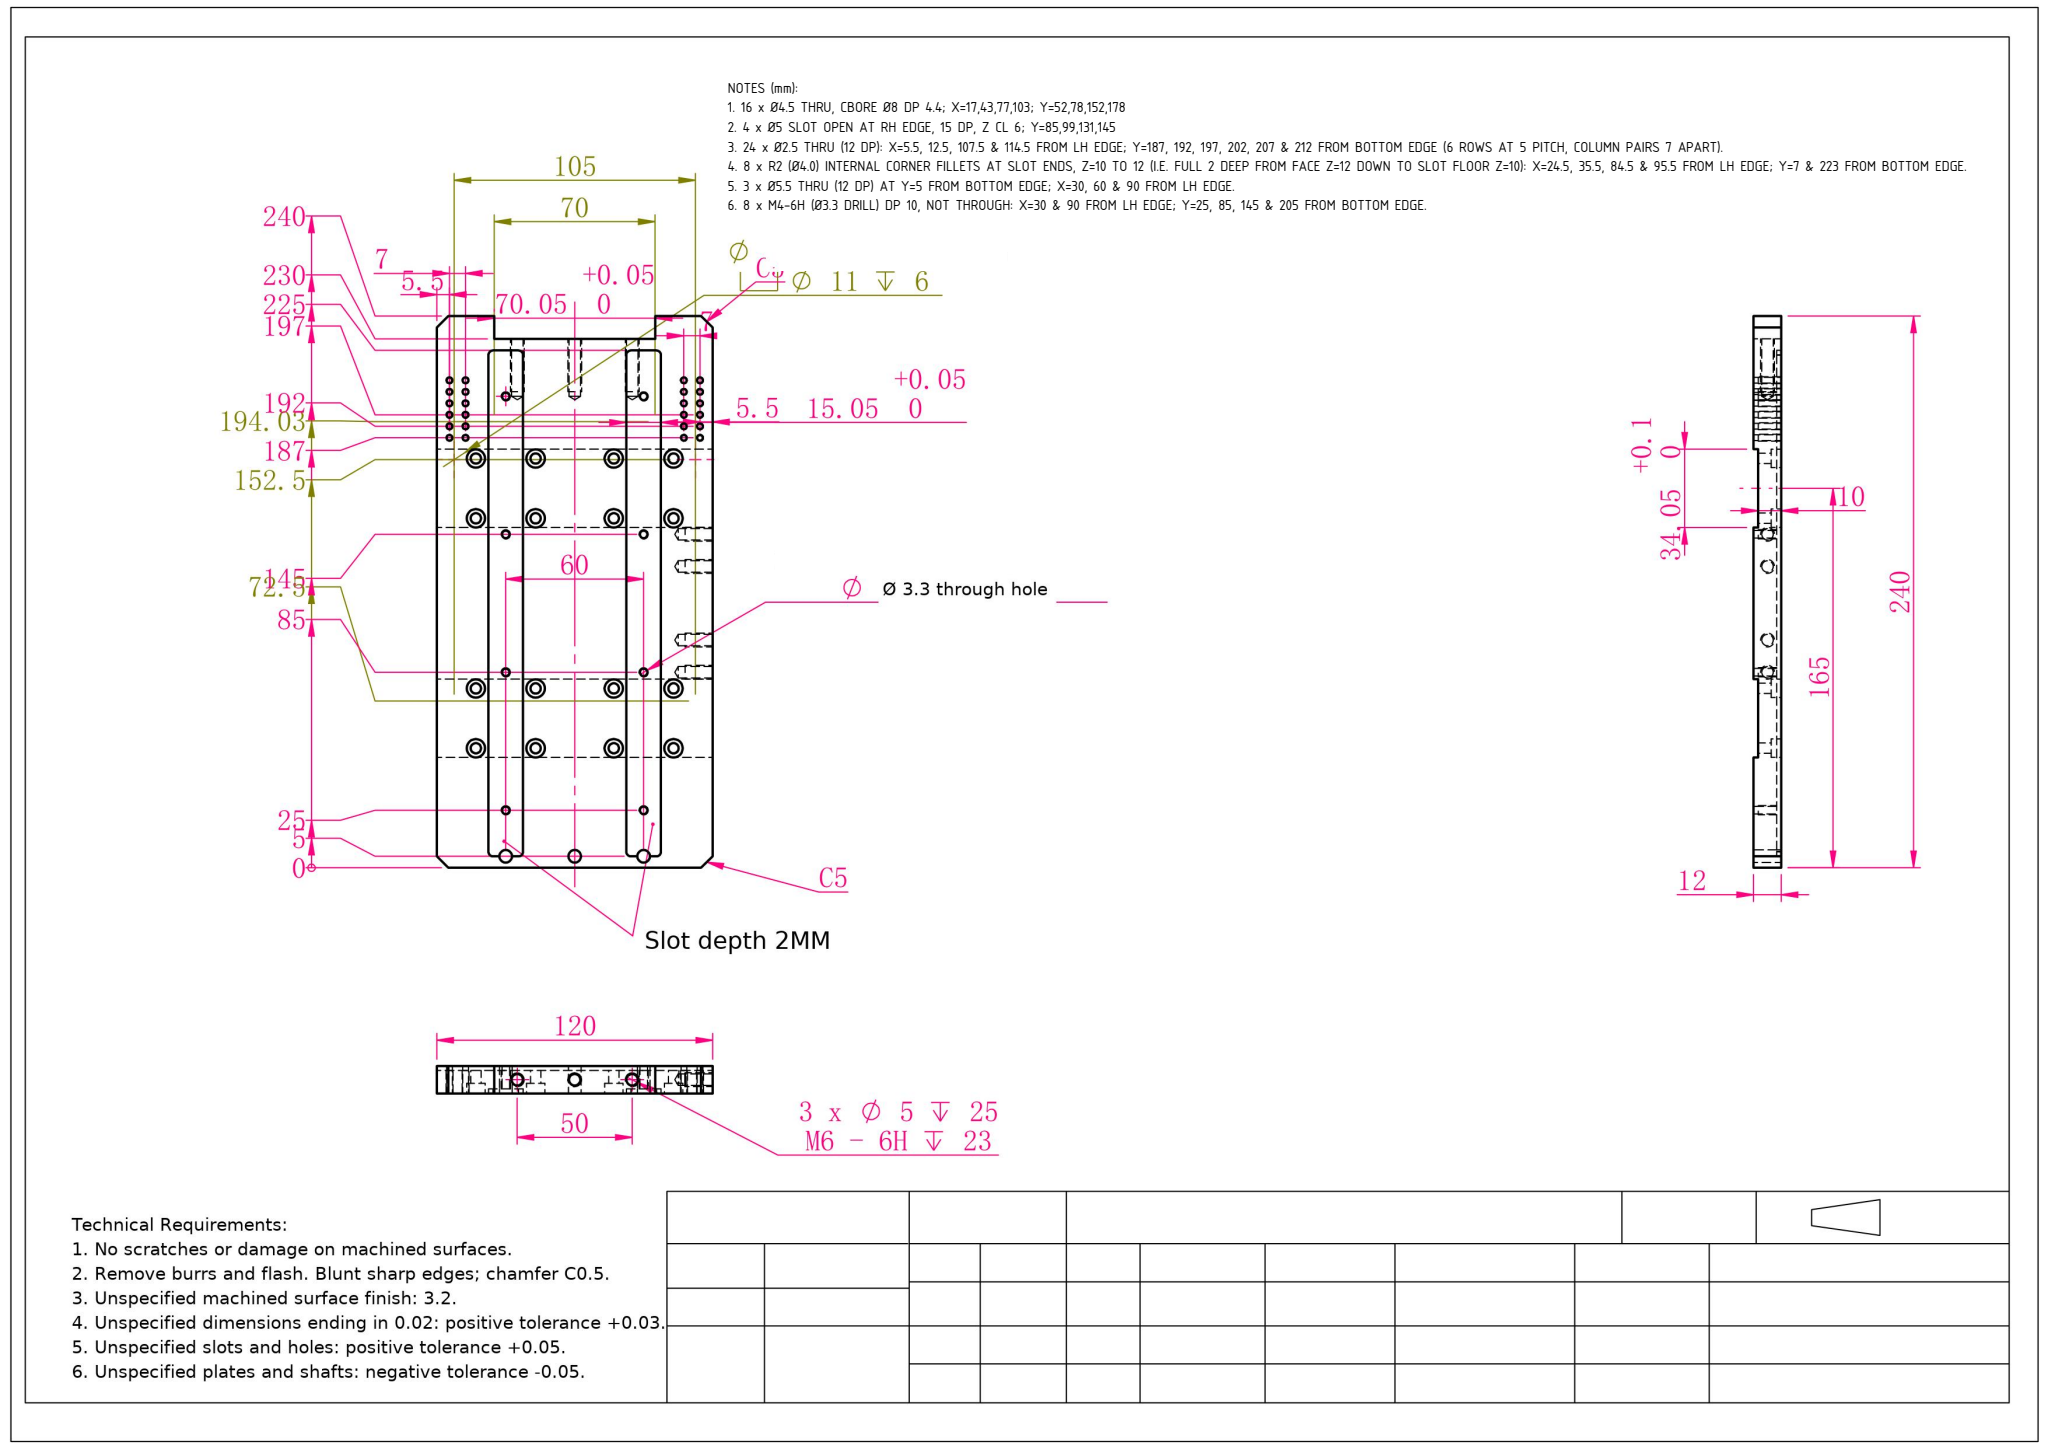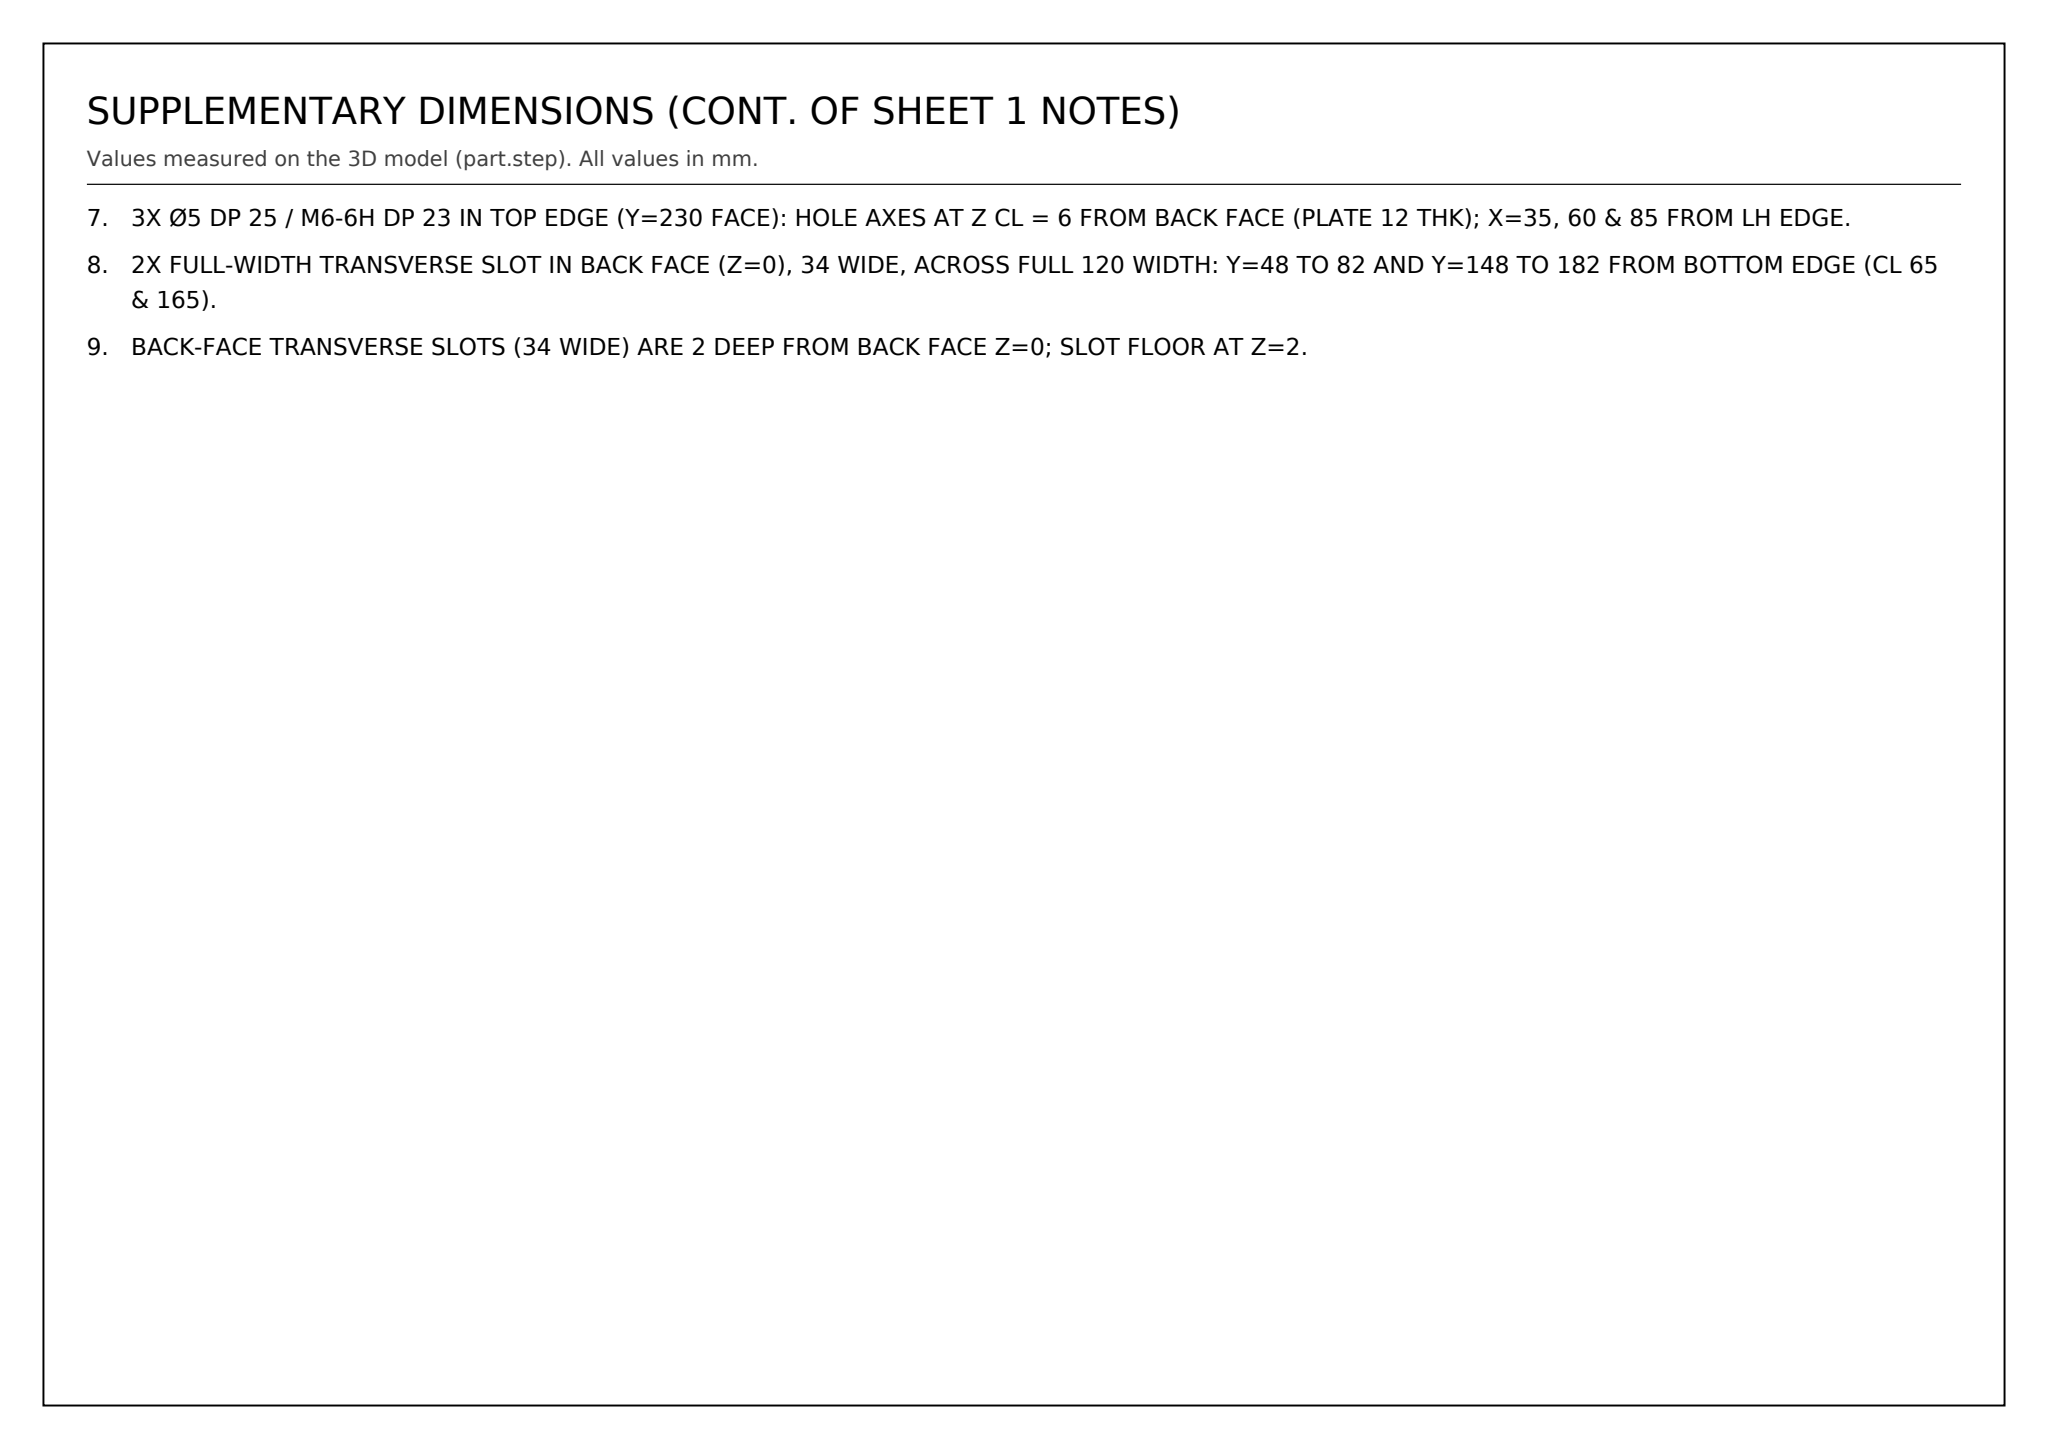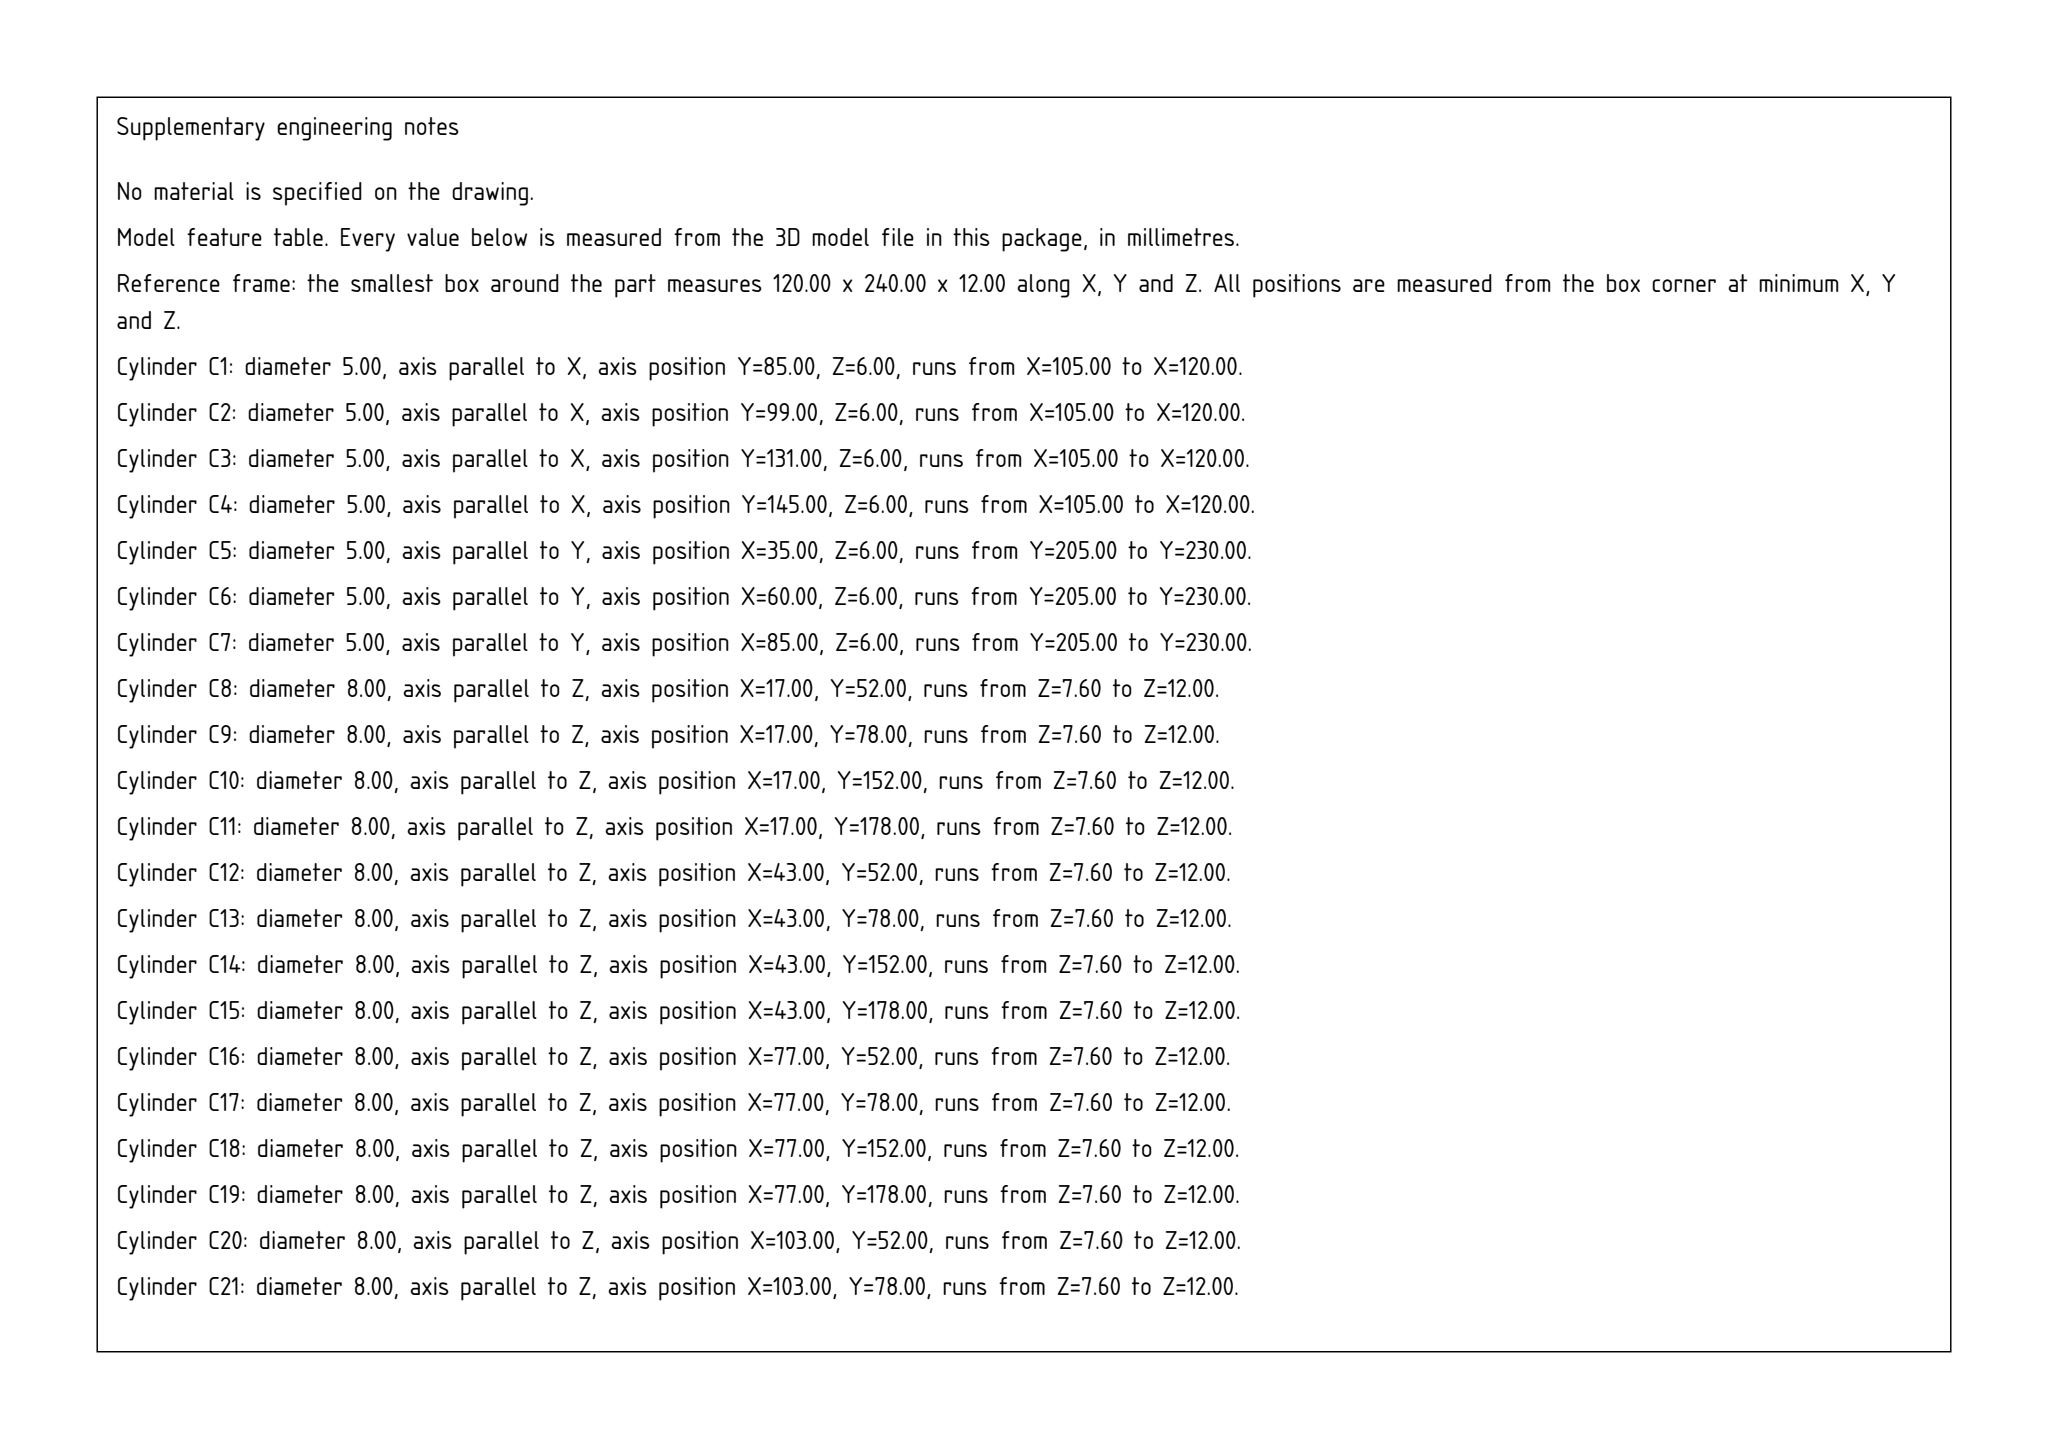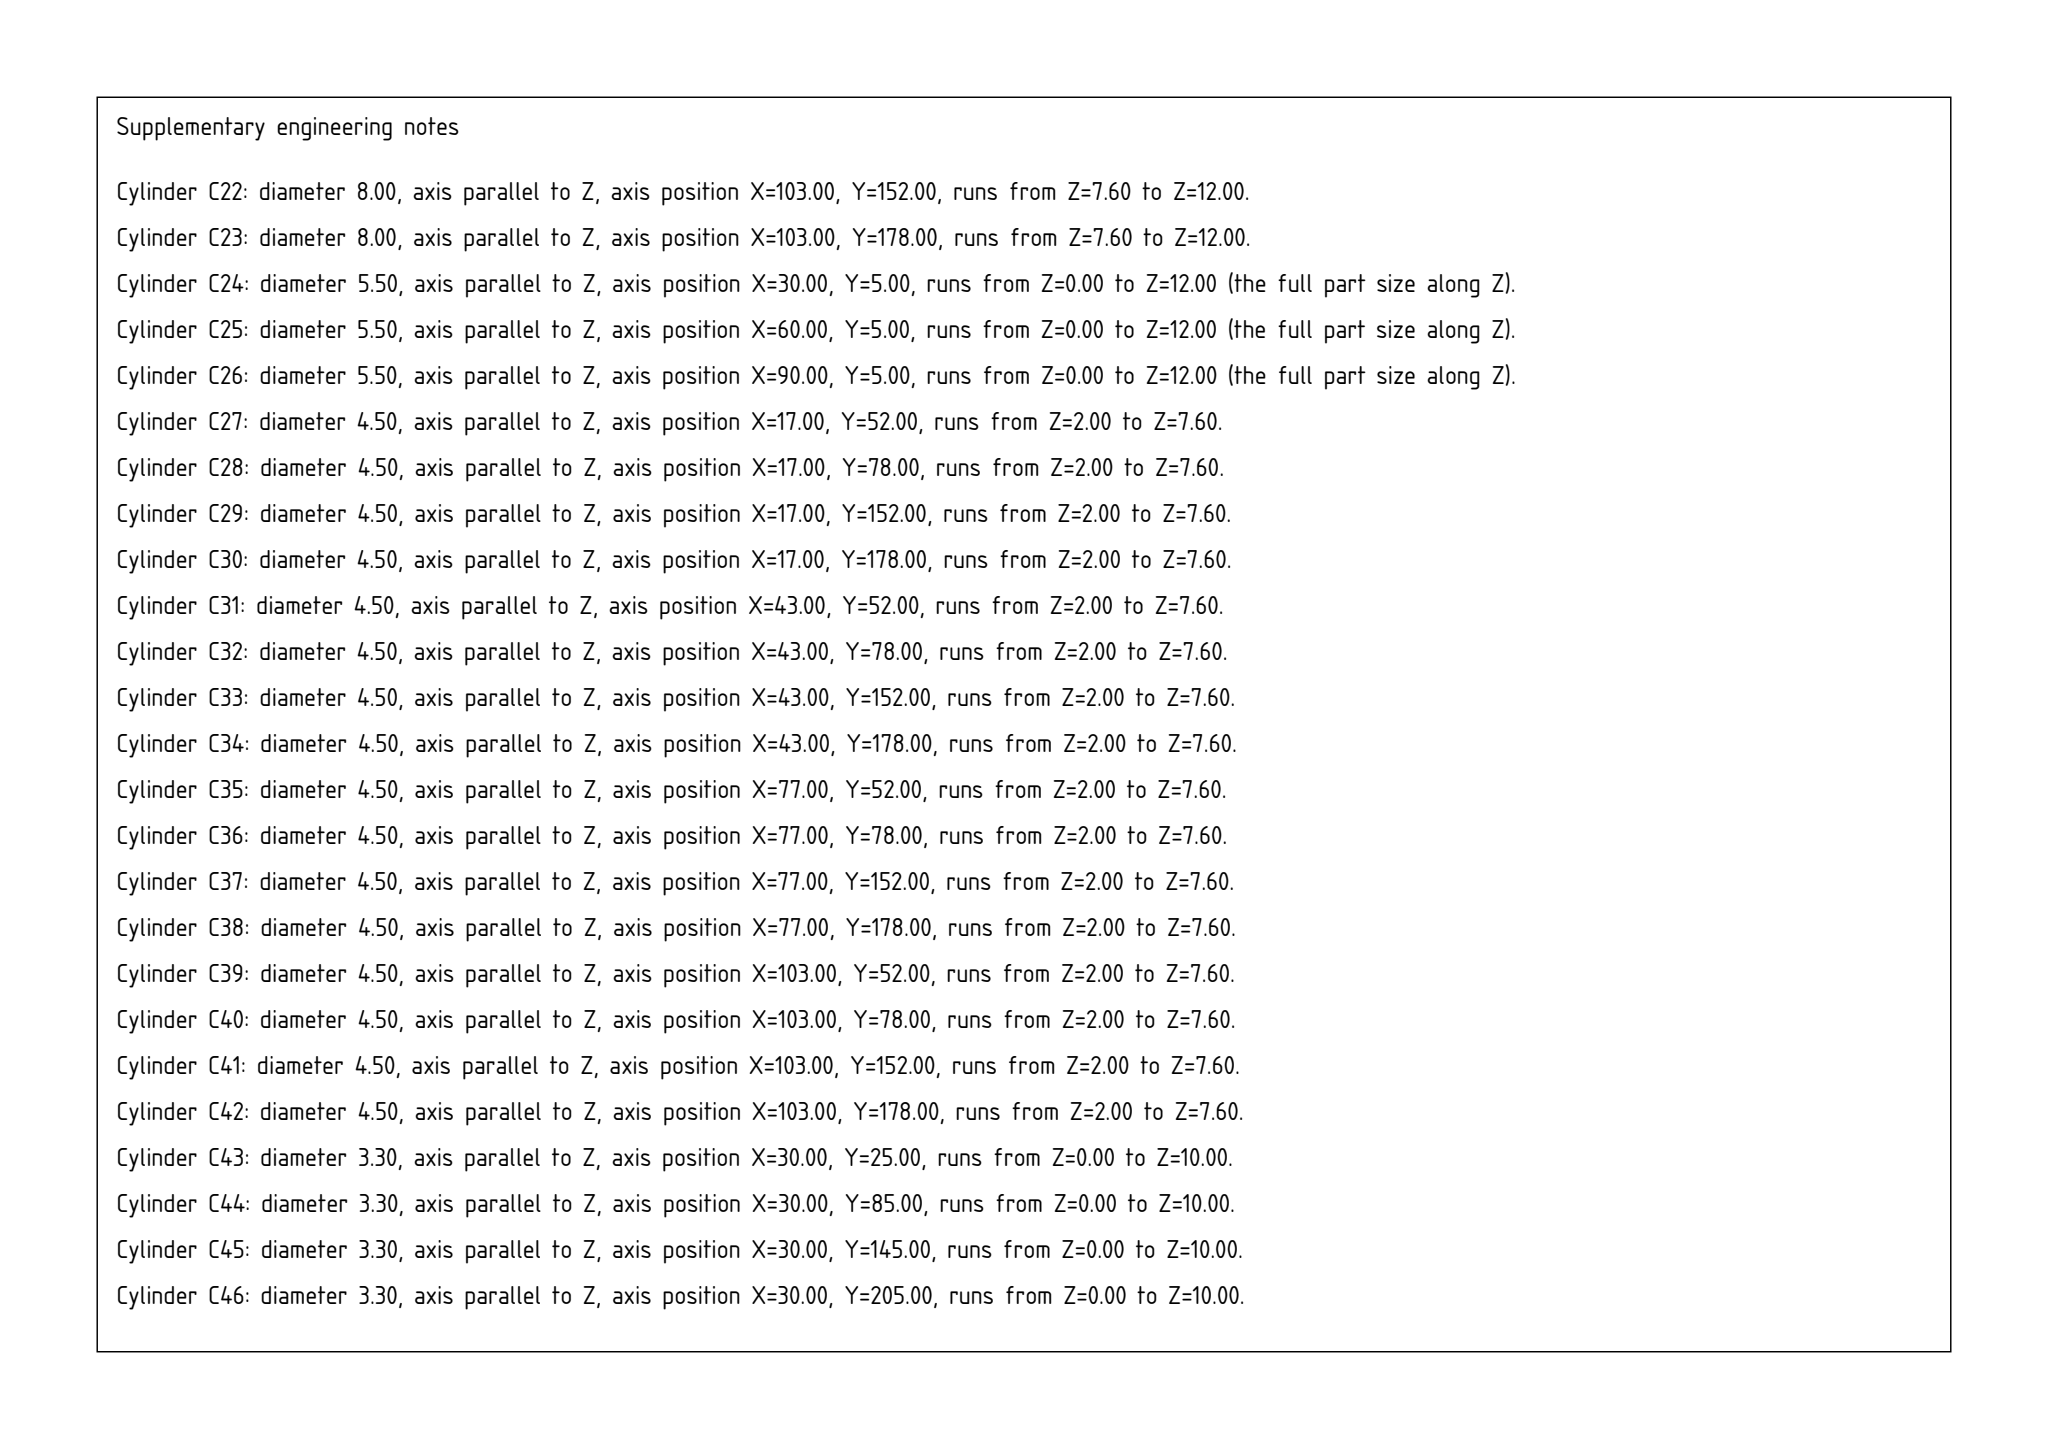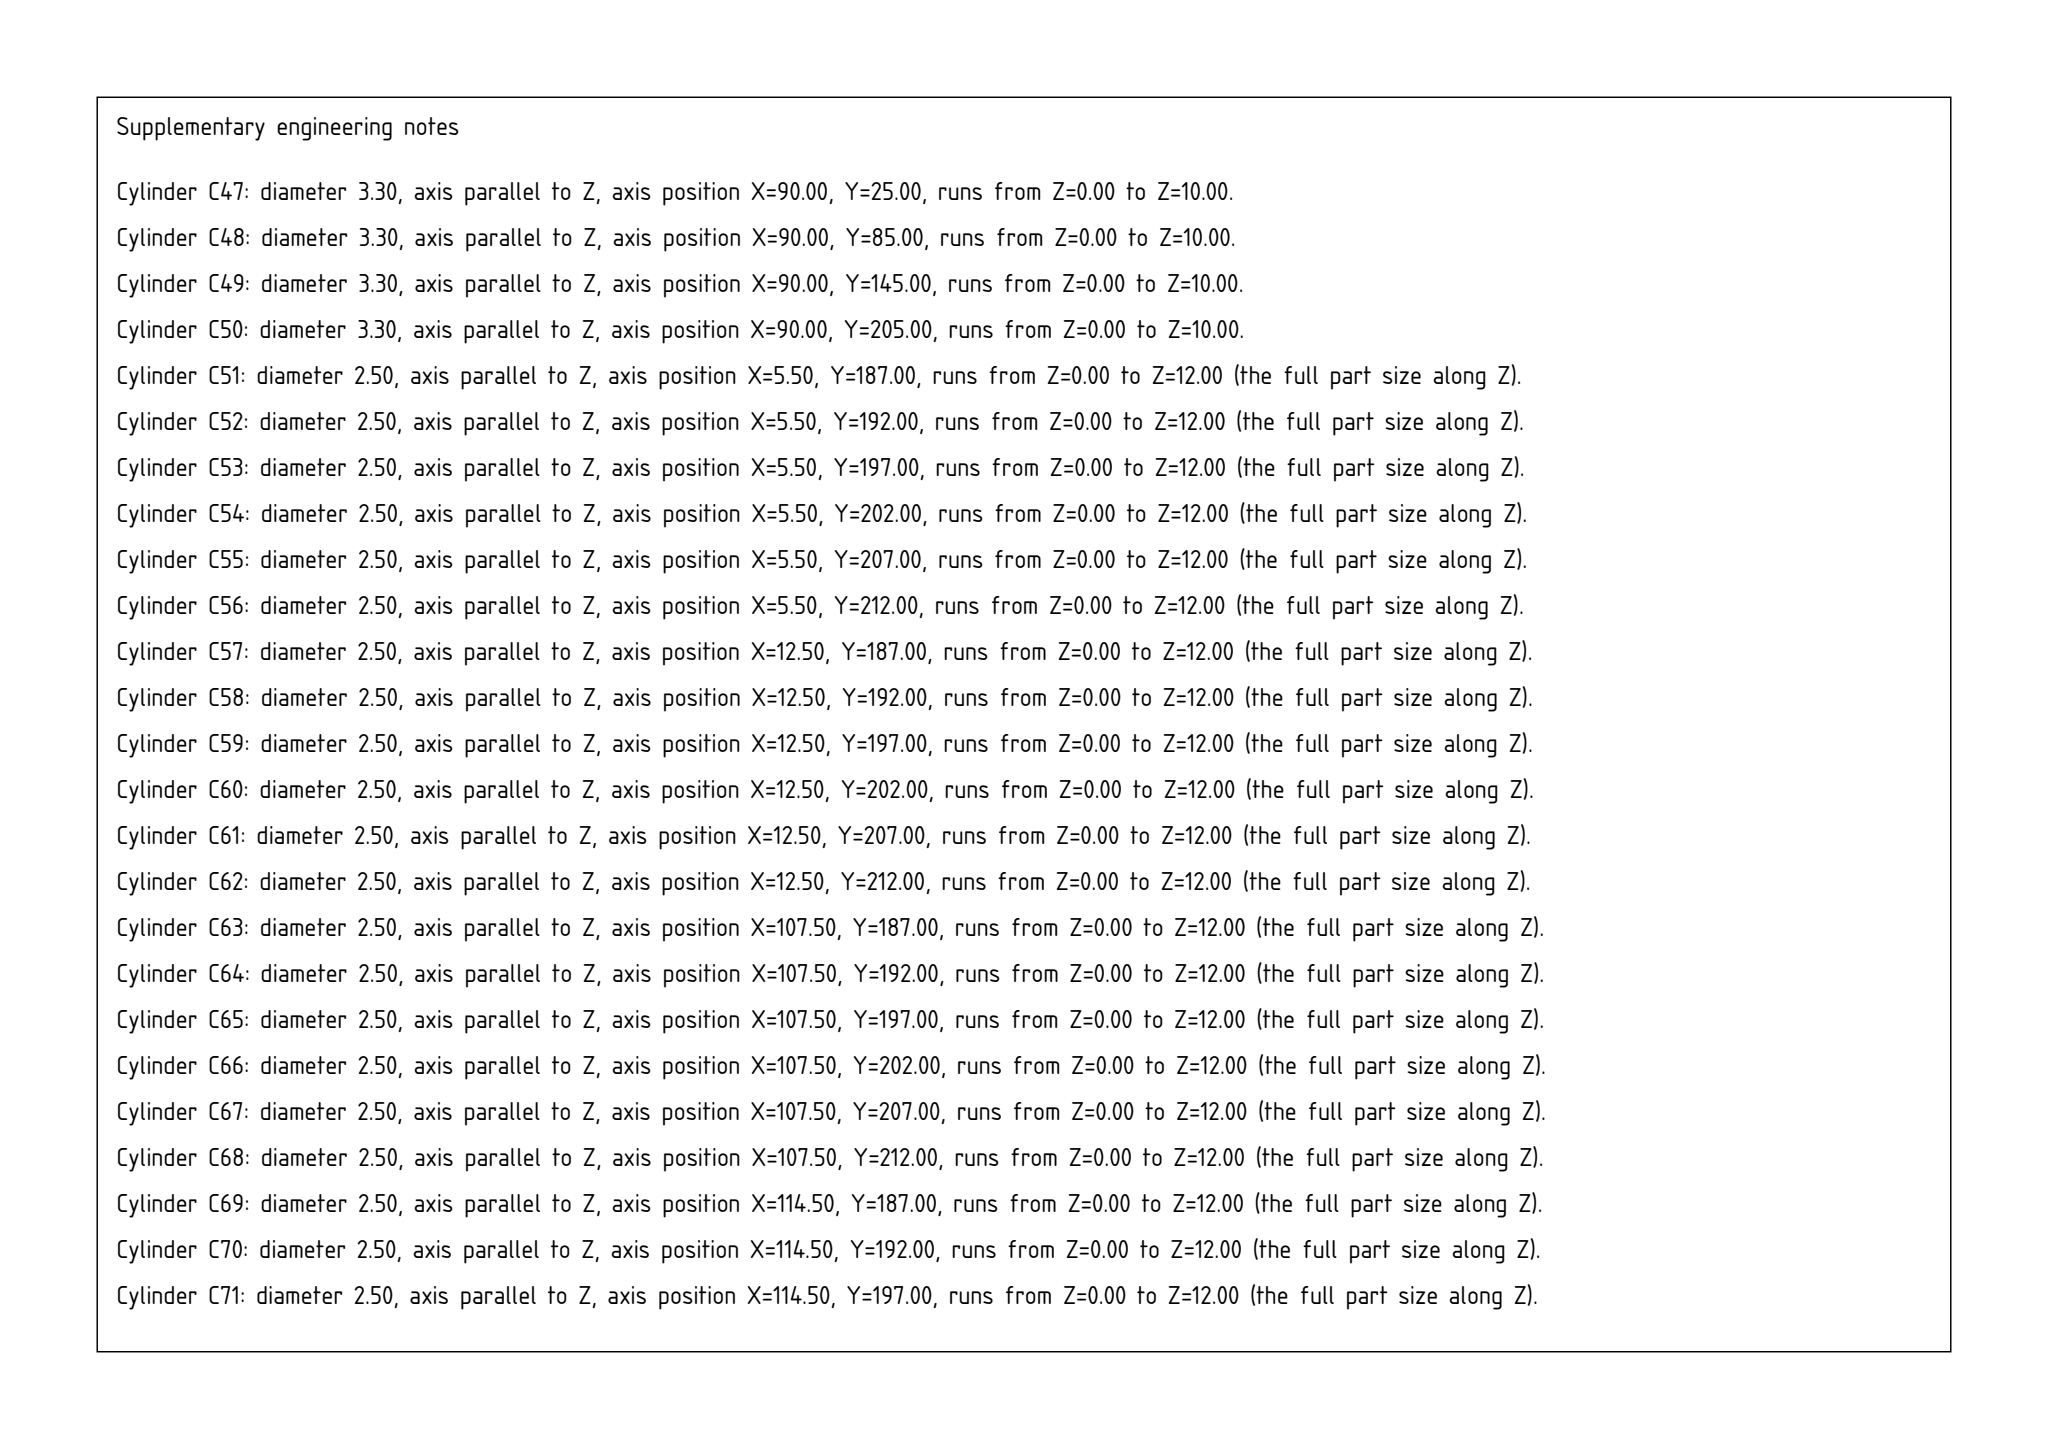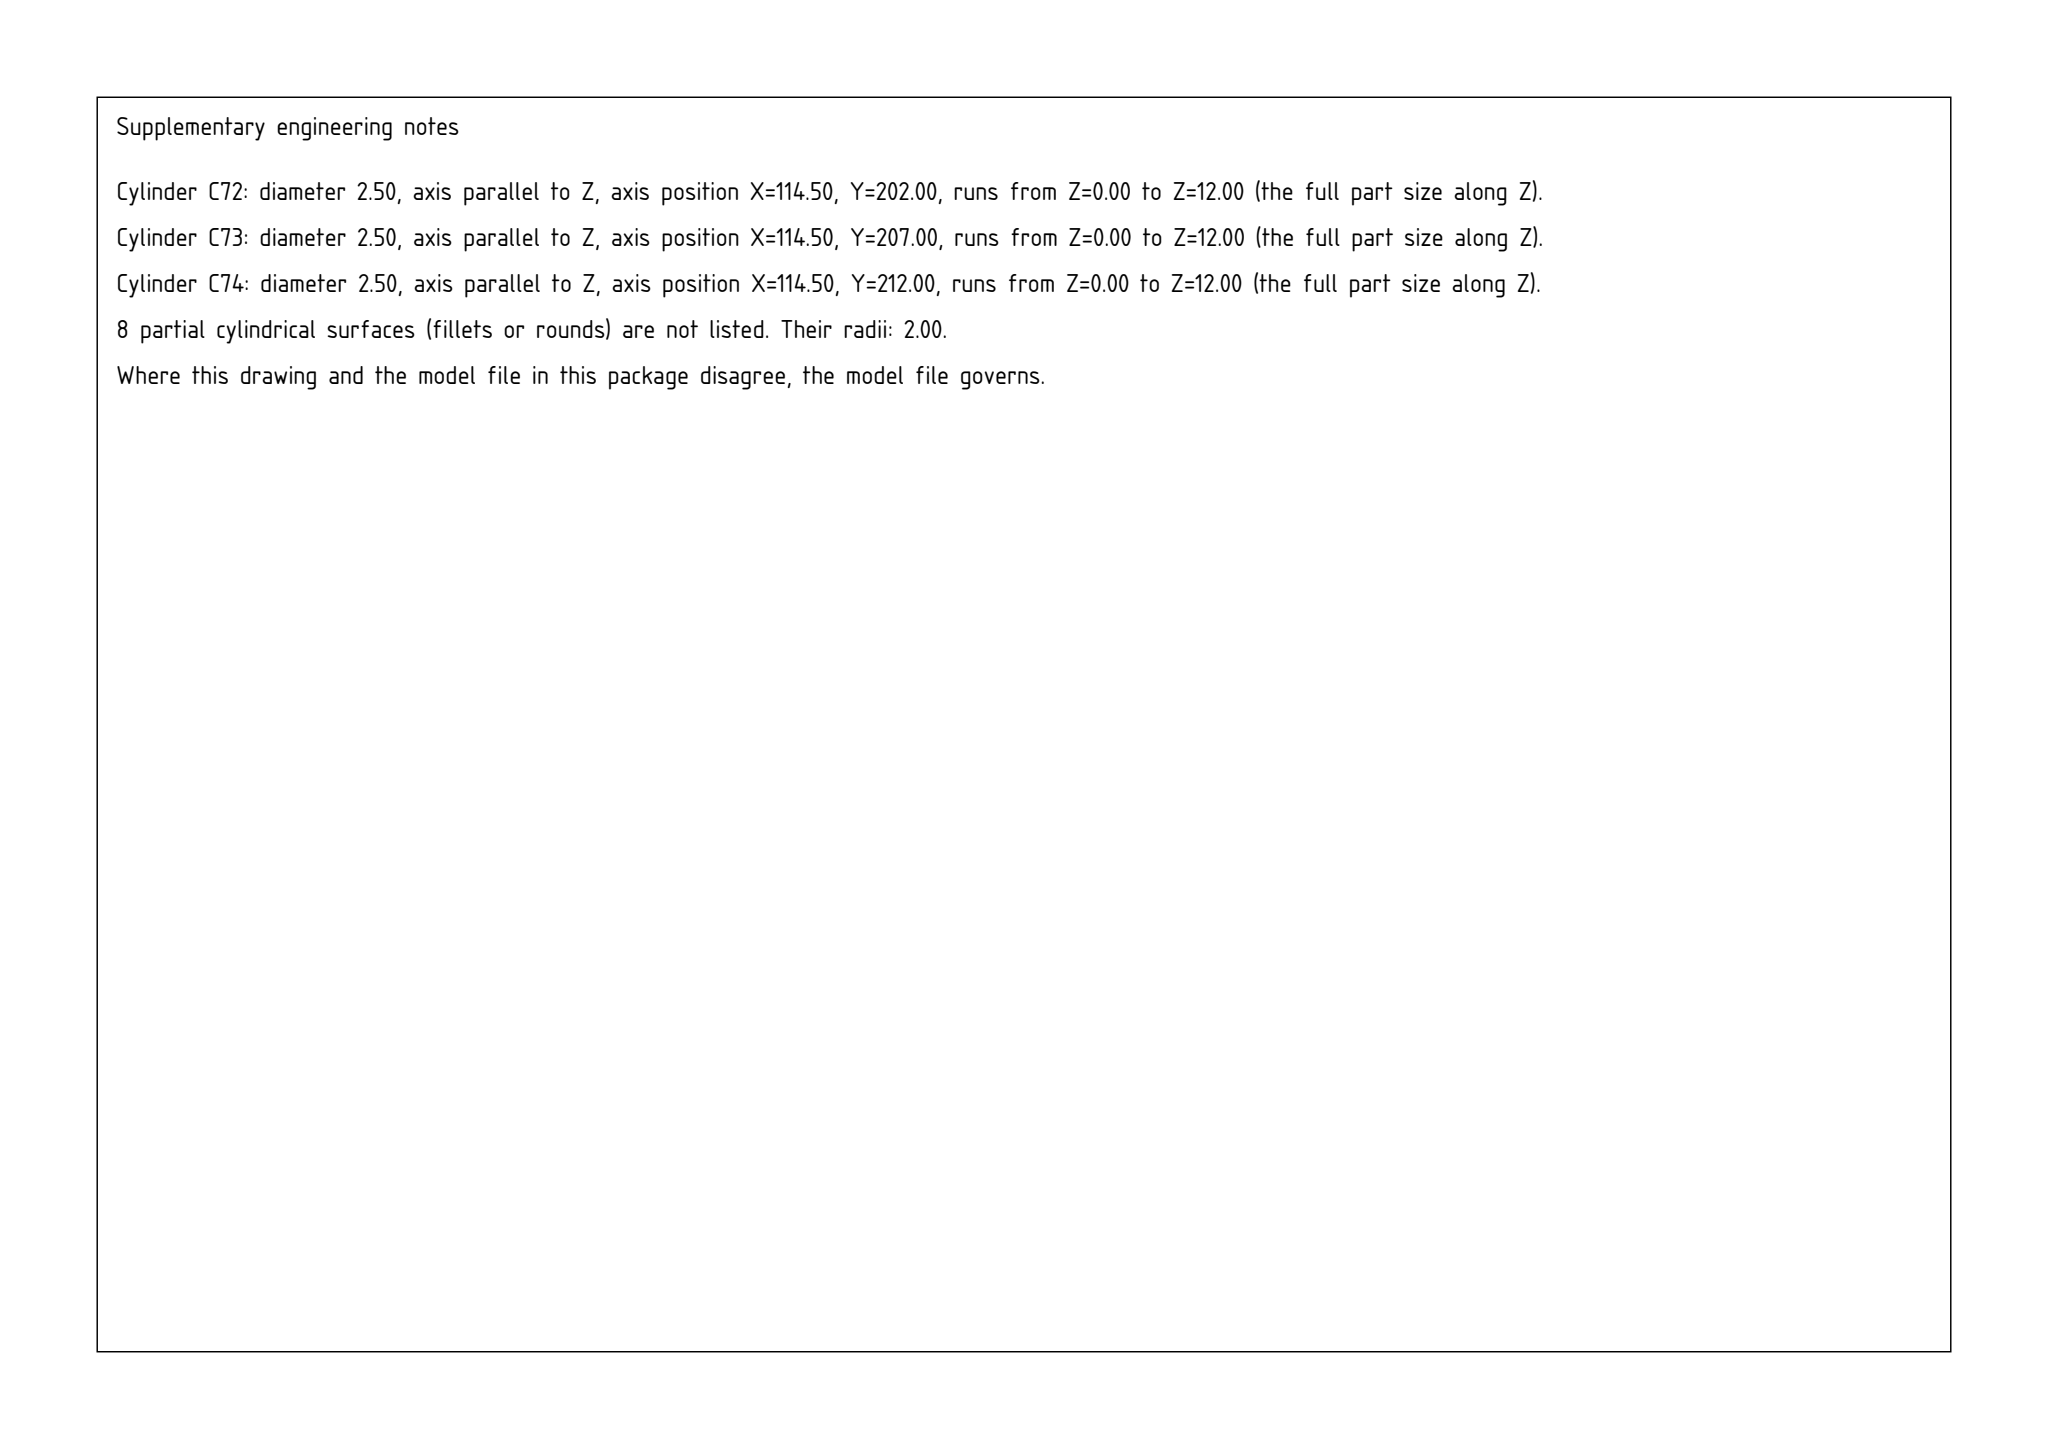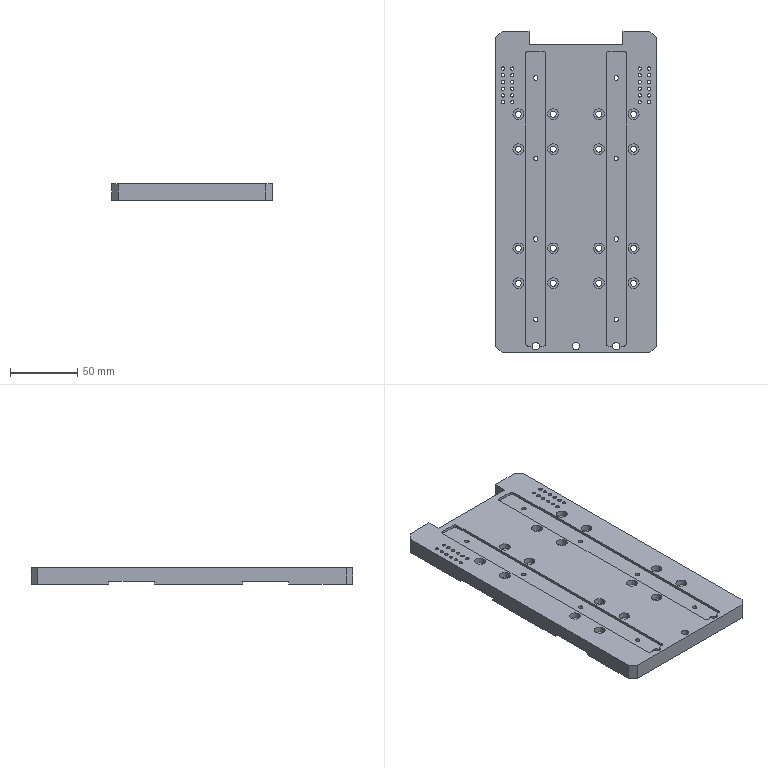Part | SolidWorks | mm | 1 solid | 220 faces | box 120 x 240 x 12 mm | volume 296431 mm3 | cylinder 156 | plane 50 | cone 14 | commonest cylinder face diameters 2.5 x48 8 x32 4.5 x32 3.3 x16 5 x14 4 x8 5.5 x6
Drawing notes:
16 x Ø4.5 THRU, CBORE Ø8 DP 4.4; X=17,43,77,103; Y=52,78,152,178 | from the solid: Cyl Ø4.5 len 5.6 with Ø8 cbore len 4.4 at x=17,43,77,103 and y=52,78,152,178
4 x Ø5 SLOT OPEN AT RH EDGE, 15 DP, Z CL 6; Y=85,99,131,145 | from the solid: Cyl Ø5 axis x len 15 at y=85,99,131,145, z=6; bbox x=120 RH edge
24 x Ø2.5 THRU (12 DP): X=5.5, 12.5, 107.5 & 114.5 FROM LH EDGE; Y=187, 192, 197, 202, 207 & 212 FROM BOTTOM EDGE (6 ROWS AT 5 PITCH, COLUMN PAIRS 7 APART). | from the solid: cylinders dia 2.5, axis z, length 12.0, pos (5.5/12.5/107.5/114.5, 187/192/197/202/207/212)
8 x R2 (Ø4.0) INTERNAL CORNER FILLETS AT SLOT ENDS, Z=10 TO 12 (I.E. FULL 2 DEEP FROM FACE Z=12 DOWN TO SLOT FLOOR Z=10): X=24.5, 35.5, 84.5 & 95.5 FROM LH EDGE; Y=7 & 223 FROM BOTTOM EDGE. | from the solid: cylinders dia 4.0, axis z, 90 deg arcs at (24.5,7),(24.5,223),(35.5,7),(35.5,223),(84.5,7),(84.5,223),(95.5,7),(95.5,223), each from z=10 to z=12; slot floor plane z=10, face z=12
3 x Ø5.5 THRU (12 DP) AT Y=5 FROM BOTTOM EDGE; X=30, 60 & 90 FROM LH EDGE. | from the solid: hole dia 5.5 axis z at (60,5) from z=0 to 12 (360 deg); at (30,5) and (90,5) dia 5.5 180 deg arcs z=0 to 10 and z=0 to 12 (half removed by slot floor at z=10) - full through hole, no stepped larger bore in model
8 x M4-6H (Ø3.3 DRILL) DP 10, NOT THROUGH: X=30 & 90 FROM LH EDGE; Y=25, 85, 145 & 205 FROM BOTTOM EDGE. | from the solid: cylinders dia 3.3, axis z, length 10.0, pos (30 & 90, 25/85/145/205)
3X Ø5 DP 25 / M6-6H DP 23 IN TOP EDGE (Y=230 FACE): HOLE AXES AT Z CL = 6 FROM BACK FACE (PLATE 12 THK); X=35, 60 & 85 FROM LH EDGE. | from the solid: Ø5 cylinders with axis y at (x=35, z=6), (x=60, z=6), (x=85, z=6), each running from y=205 to y=230, i.e. 25 deep into the y=230 edge face (plane y=230, extent x 25-95, z 0-12); bottom edge is y=0 (plane y=0, x 5-115).
2X FULL-WIDTH TRANSVERSE SLOT IN BACK FACE (Z=0), 34 WIDE, ACROSS FULL 120 WIDTH: Y=48 TO 82 AND Y=148 TO 182 FROM BOTTOM EDGE (CL 65 & 165). | from the solid: axis_planes y=48, y=82, y=148, y=182 each extent x[0,120], z[0,2]; floor planes z=2 extent x[0,120], y[48,82] and y[148,182]
BACK-FACE TRANSVERSE SLOTS (34 WIDE) ARE 2 DEEP FROM BACK FACE Z=0; SLOT FLOOR AT Z=2. | from the solid: axis_plane z=2.0 extent x[0,120] y[48,82] and y[148,182] (floor), back face z=0 planes split at y=48/82/148/182
build123d program:
from build123d import *

# Parameters (mm, degrees)
SKETCH1_W                                       = 120
SKETCH1_H                                       = 240
BOSS_EXTRUDE1_DEPTH                             = 12
M4_TAPPED_HOLE1_D                               = 3.3
SKETCH13_W                                      = 15.05
SKETCH13_H                                      = 220
CUT_EXTRUDE1_DEPTH                              = 2
SKETCH14_W                                      = 70.05
SKETCH14_H                                      = 10
CUT_EXTRUDE2_DEPTH                              = 135.7
M6_TAPPED_HOLE1_D                               = 5
M6_TAPPED_HOLE1_DEPTH                           = 25
M6_TAPPED_HOLE1_TIP                             = 1.502
FILLET1_R                                       = 2
M5_CLEARANCE_HOLE_1_D                           = 5.5
M3_TAPPED_HOLE1_D                               = 2.5
LPATTERN2_COUNT                                 = 6
LPATTERN2_PITCH                                 = 5
MIRROR1_COPY_1_D                                = 2.5
MIRROR1_COPY_2_D                                = 2.5
MIRROR1_COPY_3_D                                = 2.5
MIRROR1_COPY_4_D                                = 2.5
MIRROR1_COPY_5_D                                = 2.5
SKETCH24_W                                      = 120
SKETCH24_H                                      = 34.05
CUT_EXTRUDE3_DEPTH                              = 2
M4_HEX_SOCKET_HEAD_CAP_SCREW_CBORE1_D           = 4.5
M4_HEX_SOCKET_HEAD_CAP_SCREW_CBORE1_CBORE_D     = 8
M4_HEX_SOCKET_HEAD_CAP_SCREW_CBORE1_CBORE_DEPTH = 4.4
CHAMFER1_SIZE                                   = 5
M6_TAPPED_HOLE2_D                               = 5
M6_TAPPED_HOLE2_DEPTH                           = 15
M6_TAPPED_HOLE2_TIP                             = 1.502
LPATTERN3_COUNT                                 = 2
LPATTERN3_PITCH                                 = 100


with BuildPart() as part:
    # Sketch1 → Boss-Extrude1 (new body)
    with BuildSketch(Plane.XY):
        Rectangle(SKETCH1_W, SKETCH1_H)
    extrude(amount=BOSS_EXTRUDE1_DEPTH)

    # M4 Tapped Hole1 (through all)
    with Locations(Plane.XY.offset(12)):
        with Locations((-30, 85), (30, 85), (-30, 25), (30, 25), (-30, -35), (30, -35), (-30, -95), (30, -95), (-30, -155), (30, -155), (-30, -215), (30, -215), (-30, -275), (30, -275), (-30, -335), (30, -335), (-30, -395), (30, -395)):
            Hole(M4_TAPPED_HOLE1_D / 2)

    # Sketch13 → Cut-Extrude1 (cut)
    with BuildSketch(Plane.XY.offset(12)):
        with Locations((-30, -5)):
            Rectangle(SKETCH13_W, SKETCH13_H)
        with Locations((30, -5)):
            Rectangle(SKETCH13_W, SKETCH13_H)
    extrude(amount=-CUT_EXTRUDE1_DEPTH, mode=Mode.SUBTRACT)

    # Sketch14 → Cut-Extrude2 (cut, through all)
    with BuildSketch(Plane.XY.offset(12)):
        with Locations((0, 115)):
            Rectangle(SKETCH14_W, SKETCH14_H)
    extrude(amount=-CUT_EXTRUDE2_DEPTH, mode=Mode.SUBTRACT)

    # M6 Tapped Hole1
    with Locations(Plane(origin=(0, 110, 0), x_dir=(1, 0, 0), z_dir=(0, 1, 0))):
        with Locations((-25, -6), (25, -6), (0, -6)):
            Hole(M6_TAPPED_HOLE1_D / 2, depth=M6_TAPPED_HOLE1_DEPTH)
            with Locations((0, 0, -(M6_TAPPED_HOLE1_DEPTH + M6_TAPPED_HOLE1_TIP / 2))):  # 118° drill point
                Cone(0, M6_TAPPED_HOLE1_D / 2, M6_TAPPED_HOLE1_TIP, mode=Mode.SUBTRACT)

    # Fillet1
    fillet1_edges = [part.edges().sort_by_distance(p)[0] for p in [
        (-37.525, -115, 11),
        (-37.525, 105, 11),
        (-22.475, 105, 11),
        (-22.475, -115, 11),
        (22.475, 105, 11),
        (37.525, 105, 11),
        (37.525, -115, 11),
        (22.475, -115, 11),
    ]]
    fillet(fillet1_edges, radius=FILLET1_R)

    # M5 Clearance Hole 1 (through all)
    with Locations(Plane(origin=(0, 0, 0), x_dir=(-1, 0, 0), z_dir=(0, 0, -1))):
        with Locations((-30, -115), (0, -115), (30, -115)):
            Hole(M5_CLEARANCE_HOLE_1_D / 2)

    # M3 Tapped Hole1 (through all)
    with Locations(Plane.XY.offset(12)):
        with Locations((47.5, 67), (54.5, 67)):
            m3_tapped_hole1 = Hole(M3_TAPPED_HOLE1_D / 2)

    # LPattern2: M3 Tapped Hole1 ×6
    with Locations(*[(0, i * LPATTERN2_PITCH, 0) for i in range(1, LPATTERN2_COUNT)]):
        add(m3_tapped_hole1, mode=Mode.SUBTRACT)

    # Mirror1: M3 Tapped Hole1 across plane
    add(m3_tapped_hole1.mirror(Plane(origin=(0, 0, 0), x_dir=(0, 0, 1), z_dir=(1, 0, 0))), mode=Mode.SUBTRACT)

    # Mirror1 copy 1 (through all)
    with Locations(Plane(origin=(0, 5, 12), x_dir=(-1, 0, 0), z_dir=(0, 0, 1))):
        with Locations((47.5, -67), (54.5, -67)):
            Hole(MIRROR1_COPY_1_D / 2)

    # Mirror1 copy 2 (through all)
    with Locations(Plane(origin=(0, 10, 12), x_dir=(-1, 0, 0), z_dir=(0, 0, 1))):
        with Locations((47.5, -67), (54.5, -67)):
            Hole(MIRROR1_COPY_2_D / 2)

    # Mirror1 copy 3 (through all)
    with Locations(Plane(origin=(0, 15, 12), x_dir=(-1, 0, 0), z_dir=(0, 0, 1))):
        with Locations((47.5, -67), (54.5, -67)):
            Hole(MIRROR1_COPY_3_D / 2)

    # Mirror1 copy 4 (through all)
    with Locations(Plane(origin=(0, 20, 12), x_dir=(-1, 0, 0), z_dir=(0, 0, 1))):
        with Locations((47.5, -67), (54.5, -67)):
            Hole(MIRROR1_COPY_4_D / 2)

    # Mirror1 copy 5 (through all)
    with Locations(Plane(origin=(0, 25, 12), x_dir=(-1, 0, 0), z_dir=(0, 0, 1))):
        with Locations((47.5, -67), (54.5, -67)):
            Hole(MIRROR1_COPY_5_D / 2)

    # Sketch24 → Cut-Extrude3 (cut)
    with BuildSketch(Plane(origin=(0, 0, 0), x_dir=(-1, 0, 0), z_dir=(0, 0, -1))):
        with Locations((0, 45)):
            Rectangle(SKETCH24_W, SKETCH24_H)
        with Locations((0, -55)):
            Rectangle(SKETCH24_W, SKETCH24_H)
    extrude(amount=-CUT_EXTRUDE3_DEPTH, mode=Mode.SUBTRACT)

    # M4 Hex Socket Head Cap Screw CBORE1 (through all)
    with Locations(Plane.XY.offset(12)):
        with Locations((17, 58), (43, 58), (-17, 58), (-43, 58), (43, 32), (17, 32), (-43, 32), (-17, 32)):
            m4_hex_socket_head_cap_screw_cbore1 = CounterBoreHole(M4_HEX_SOCKET_HEAD_CAP_SCREW_CBORE1_D / 2, M4_HEX_SOCKET_HEAD_CAP_SCREW_CBORE1_CBORE_D / 2, M4_HEX_SOCKET_HEAD_CAP_SCREW_CBORE1_CBORE_DEPTH)

    # Chamfer1
    chamfer1_edges = [part.edges().sort_by_distance(p)[0] for p in [
        (60, 120, 6),
        (60, -120, 6),
        (-60, -120, 6),
        (-60, 120, 6),
    ]]
    chamfer(chamfer1_edges, length=CHAMFER1_SIZE)

    # M6 Tapped Hole2
    with Locations(Plane(origin=(60, 0, 0), x_dir=(0, 0, -1), z_dir=(1, 0, 0))):
        with Locations((-6, -21), (-6, -35), (-6, 25), (-6, 11)):
            Hole(M6_TAPPED_HOLE2_D / 2, depth=M6_TAPPED_HOLE2_DEPTH)
            with Locations((0, 0, -(M6_TAPPED_HOLE2_DEPTH + M6_TAPPED_HOLE2_TIP / 2))):  # 118° drill point
                Cone(0, M6_TAPPED_HOLE2_D / 2, M6_TAPPED_HOLE2_TIP, mode=Mode.SUBTRACT)

    # LPattern3: M4 Hex Socket Head Cap Screw CBORE1 ×2
    with Locations(*[(0, -i * LPATTERN3_PITCH, 0) for i in range(1, LPATTERN3_COUNT)]):
        add(m4_hex_socket_head_cap_screw_cbore1, mode=Mode.SUBTRACT)


solid = part.part